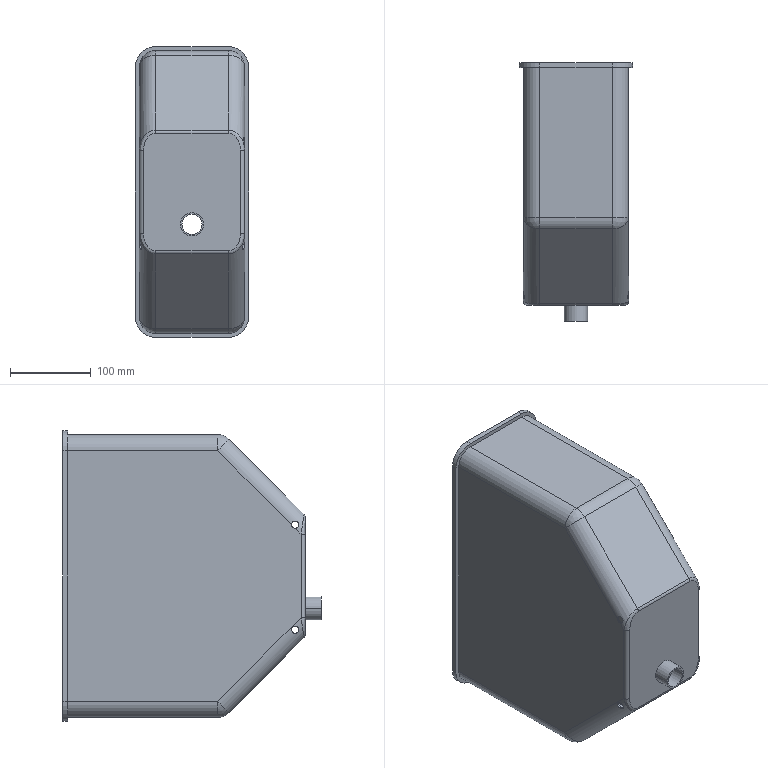Component | SolidWorks | SeedBox-1 | 1 solid | 90 faces | volume 576208 mm3 | cylinder 48 | plane 26 | spline 8 | sphere 8 | commonest cylinder face diameters 40 x10 36 x10 9 x8 10 x4 50 x4 6 x4 46 x4 29 x2